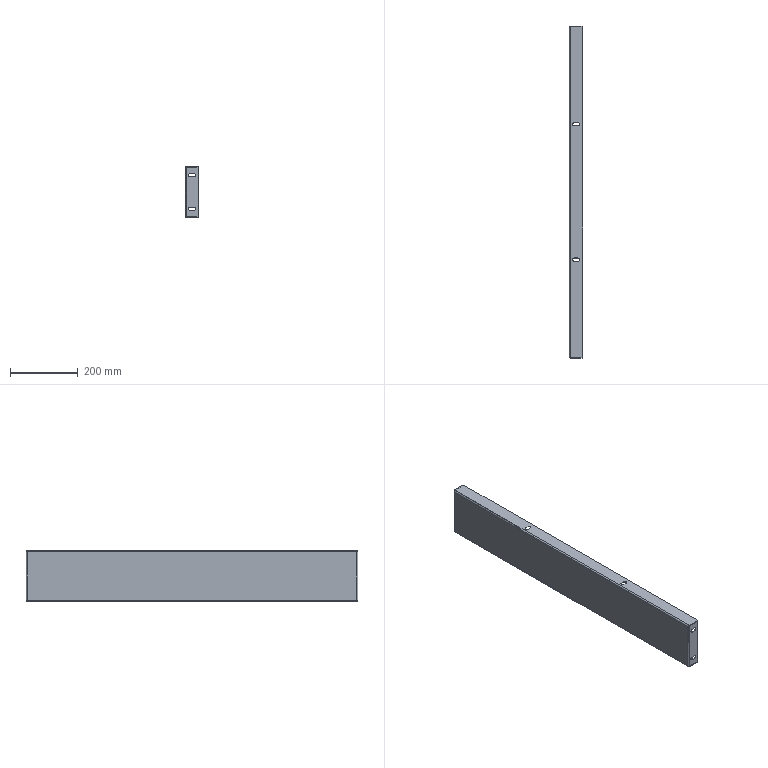Component | SolidWorks | FrontBeam-1 | 1 solid | 86 faces | volume 455096 mm3 | plane 46 | cylinder 32 | spline 8 | commonest cylinder face diameters 10 x24 8 x4 4 x4 | material Plain Carbon Steel